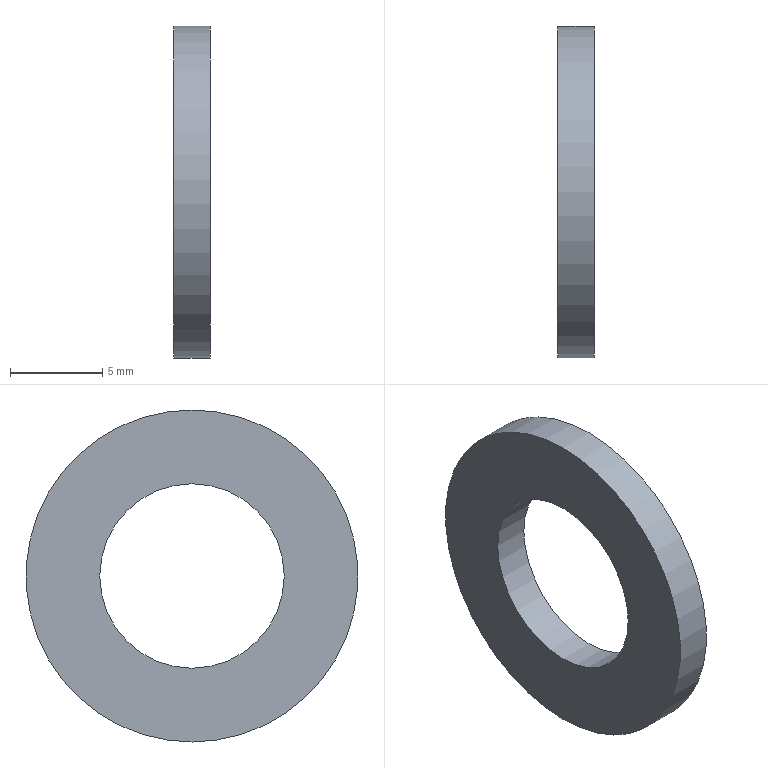Component | NX | CCJ-025 | 1 solid | 4 faces | box 2 x 18 x 18 mm | volume 352 mm3 | plane 2 | cylinder 2 | commonest cylinder face diameters 18 x1 10 x1
STEP:
#1=CARTESIAN_POINT('',(0.,0.,0.));
#2=DIRECTION('',(0.,0.,1.));
#3=DIRECTION('',(1.,0.,0.));
#4=AXIS2_PLACEMENT_3D('',#1,#2,#3);
#5=CARTESIAN_POINT('',(-40.,53.506,-47.227));
#6=VERTEX_POINT('',#5);
#7=CARTESIAN_POINT('',(-40.,53.506,-56.227));
#8=DIRECTION('',(-1.,0.,0.));
#9=DIRECTION('',(0.,0.,1.));
#10=AXIS2_PLACEMENT_3D('',#7,#8,#9);
#11=CIRCLE('',#10,9.);
#12=CARTESIAN_POINT('',(-40.,53.506,-56.227));
#13=DIRECTION('',(1.,0.,0.));
#14=DIRECTION('',(0.,0.,-1.));
#15=AXIS2_PLACEMENT_3D('',#12,#13,#14);
#16=PLANE('',#15);
#17=CARTESIAN_POINT('',(-9.,0.));
#18=CARTESIAN_POINT('',(-9.,15.588));
#19=CARTESIAN_POINT('',(4.5,7.794));
#20=CARTESIAN_POINT('',(18.,0.));
#21=CARTESIAN_POINT('',(4.5,-7.794));
#22=CARTESIAN_POINT('',(-9.,-15.588));
#23=CARTESIAN_POINT('',(-9.,0.));
#24=(BOUNDED_CURVE()B_SPLINE_CURVE(2,(#17,#18,#19,#20,#21,#22,#23),.UNSPECIFIED.,.T.,.F.)B_SPLINE_CURVE_WITH_KNOTS((1,2,2,2,2,1),(-2.094,0.,2.094,4.189,6.283,8.378),.UNSPECIFIED.)CURVE()GEOMETRIC_REPRESENTATION_ITEM()RATIONAL_B_SPLINE_CURVE((1.,0.5,1.,0.5,1.,0.5,1.))REPRESENTATION_ITEM(''));
#25=(GEOMETRIC_REPRESENTATION_CONTEXT(2)PARAMETRIC_REPRESENTATION_CONTEXT()REPRESENTATION_CONTEXT('',''));
#26=DEFINITIONAL_REPRESENTATION('',(#24),#25);
#27=PCURVE('',#16,#26);
#28=CARTESIAN_POINT('',(-40.,53.506,-56.227));
#29=DIRECTION('',(-1.,0.,0.));
#30=DIRECTION('',(0.,0.,1.));
#31=AXIS2_PLACEMENT_3D('',#28,#29,#30);
#32=CYLINDRICAL_SURFACE('',#31,9.);
#33=CARTESIAN_POINT('',(0.,0.));
#34=DIRECTION('',(1.,0.));
#35=VECTOR('',#34,1.);
#36=LINE('',#33,#35);
#37=(GEOMETRIC_REPRESENTATION_CONTEXT(2)PARAMETRIC_REPRESENTATION_CONTEXT()REPRESENTATION_CONTEXT('',''));
#38=DEFINITIONAL_REPRESENTATION('',(#36),#37);
#39=PCURVE('',#32,#38);
#40=SURFACE_CURVE('',#11,(#27,#39),.PCURVE_S1.);
#41=EDGE_CURVE('',#6,#6,#40,.T.);
#42=ORIENTED_EDGE('',*,*,#41,.F.);
#43=EDGE_LOOP('',(#42));
#44=FACE_BOUND('',#43,.T.);
#45=CARTESIAN_POINT('',(-40.,53.506,-51.227));
#46=VERTEX_POINT('',#45);
#47=CARTESIAN_POINT('',(-40.,53.506,-56.227));
#48=DIRECTION('',(-1.,0.,0.));
#49=DIRECTION('',(0.,0.,1.));
#50=AXIS2_PLACEMENT_3D('',#47,#48,#49);
#51=CIRCLE('',#50,5.);
#52=CARTESIAN_POINT('',(-5.,0.));
#53=CARTESIAN_POINT('',(-5.,8.66));
#54=CARTESIAN_POINT('',(2.5,4.33));
#55=CARTESIAN_POINT('',(10.,0.));
#56=CARTESIAN_POINT('',(2.5,-4.33));
#57=CARTESIAN_POINT('',(-5.,-8.66));
#58=CARTESIAN_POINT('',(-5.,0.));
#59=(BOUNDED_CURVE()B_SPLINE_CURVE(2,(#52,#53,#54,#55,#56,#57,#58),.UNSPECIFIED.,.T.,.F.)B_SPLINE_CURVE_WITH_KNOTS((1,2,2,2,2,1),(-2.094,0.,2.094,4.189,6.283,8.378),.UNSPECIFIED.)CURVE()GEOMETRIC_REPRESENTATION_ITEM()RATIONAL_B_SPLINE_CURVE((1.,0.5,1.,0.5,1.,0.5,1.))REPRESENTATION_ITEM(''));
#60=(GEOMETRIC_REPRESENTATION_CONTEXT(2)PARAMETRIC_REPRESENTATION_CONTEXT()REPRESENTATION_CONTEXT('',''));
#61=DEFINITIONAL_REPRESENTATION('',(#59),#60);
#62=PCURVE('',#16,#61);
#63=CARTESIAN_POINT('',(-40.,53.506,-56.227));
#64=DIRECTION('',(-1.,0.,0.));
#65=DIRECTION('',(0.,0.,1.));
#66=AXIS2_PLACEMENT_3D('',#63,#64,#65);
#67=CYLINDRICAL_SURFACE('',#66,5.);
#68=CARTESIAN_POINT('',(0.,0.));
#69=DIRECTION('',(1.,0.));
#70=VECTOR('',#69,1.);
#71=LINE('',#68,#70);
#72=(GEOMETRIC_REPRESENTATION_CONTEXT(2)PARAMETRIC_REPRESENTATION_CONTEXT()REPRESENTATION_CONTEXT('',''));
#73=DEFINITIONAL_REPRESENTATION('',(#71),#72);
#74=PCURVE('',#67,#73);
#75=SURFACE_CURVE('',#51,(#62,#74),.PCURVE_S1.);
#76=EDGE_CURVE('',#46,#46,#75,.T.);
#77=ORIENTED_EDGE('',*,*,#76,.T.);
#78=EDGE_LOOP('',(#77));
#79=FACE_BOUND('',#78,.T.);
#80=ADVANCED_FACE('',(#44,#79),#16,.T.);
#81=CARTESIAN_POINT('',(-42.,53.506,-47.227));
#82=VERTEX_POINT('',#81);
#83=CARTESIAN_POINT('',(-42.,53.506,-56.227));
#84=DIRECTION('',(-1.,0.,0.));
#85=DIRECTION('',(0.,0.,1.));
#86=AXIS2_PLACEMENT_3D('',#83,#84,#85);
#87=CIRCLE('',#86,9.);
#88=CARTESIAN_POINT('',(-42.,53.506,-56.227));
#89=DIRECTION('',(1.,0.,0.));
#90=DIRECTION('',(0.,0.,-1.));
#91=AXIS2_PLACEMENT_3D('',#88,#89,#90);
#92=PLANE('',#91);
#93=CARTESIAN_POINT('',(-9.,0.));
#94=CARTESIAN_POINT('',(-9.,15.588));
#95=CARTESIAN_POINT('',(4.5,7.794));
#96=CARTESIAN_POINT('',(18.,0.));
#97=CARTESIAN_POINT('',(4.5,-7.794));
#98=CARTESIAN_POINT('',(-9.,-15.588));
#99=CARTESIAN_POINT('',(-9.,0.));
#100=(BOUNDED_CURVE()B_SPLINE_CURVE(2,(#93,#94,#95,#96,#97,#98,#99),.UNSPECIFIED.,.T.,.F.)B_SPLINE_CURVE_WITH_KNOTS((1,2,2,2,2,1),(-2.094,0.,2.094,4.189,6.283,8.378),.UNSPECIFIED.)CURVE()GEOMETRIC_REPRESENTATION_ITEM()RATIONAL_B_SPLINE_CURVE((1.,0.5,1.,0.5,1.,0.5,1.))REPRESENTATION_ITEM(''));
#101=(GEOMETRIC_REPRESENTATION_CONTEXT(2)PARAMETRIC_REPRESENTATION_CONTEXT()REPRESENTATION_CONTEXT('',''));
#102=DEFINITIONAL_REPRESENTATION('',(#100),#101);
#103=PCURVE('',#92,#102);
#104=CARTESIAN_POINT('',(0.,2.));
#105=DIRECTION('',(1.,0.));
#106=VECTOR('',#105,1.);
#107=LINE('',#104,#106);
#108=(GEOMETRIC_REPRESENTATION_CONTEXT(2)PARAMETRIC_REPRESENTATION_CONTEXT()REPRESENTATION_CONTEXT('',''));
#109=DEFINITIONAL_REPRESENTATION('',(#107),#108);
#110=PCURVE('',#32,#109);
#111=SURFACE_CURVE('',#87,(#103,#110),.PCURVE_S1.);
#112=EDGE_CURVE('',#82,#82,#111,.T.);
#113=ORIENTED_EDGE('',*,*,#112,.T.);
#114=EDGE_LOOP('',(#113));
#115=FACE_BOUND('',#114,.T.);
#116=CARTESIAN_POINT('',(-42.,53.506,-51.227));
#117=VERTEX_POINT('',#116);
#118=CARTESIAN_POINT('',(-42.,53.506,-56.227));
#119=DIRECTION('',(-1.,0.,0.));
#120=DIRECTION('',(0.,0.,1.));
#121=AXIS2_PLACEMENT_3D('',#118,#119,#120);
#122=CIRCLE('',#121,5.);
#123=CARTESIAN_POINT('',(-5.,0.));
#124=CARTESIAN_POINT('',(-5.,8.66));
#125=CARTESIAN_POINT('',(2.5,4.33));
#126=CARTESIAN_POINT('',(10.,0.));
#127=CARTESIAN_POINT('',(2.5,-4.33));
#128=CARTESIAN_POINT('',(-5.,-8.66));
#129=CARTESIAN_POINT('',(-5.,0.));
#130=(BOUNDED_CURVE()B_SPLINE_CURVE(2,(#123,#124,#125,#126,#127,#128,#129),.UNSPECIFIED.,.T.,.F.)B_SPLINE_CURVE_WITH_KNOTS((1,2,2,2,2,1),(-2.094,0.,2.094,4.189,6.283,8.378),.UNSPECIFIED.)CURVE()GEOMETRIC_REPRESENTATION_ITEM()RATIONAL_B_SPLINE_CURVE((1.,0.5,1.,0.5,1.,0.5,1.))REPRESENTATION_ITEM(''));
#131=(GEOMETRIC_REPRESENTATION_CONTEXT(2)PARAMETRIC_REPRESENTATION_CONTEXT()REPRESENTATION_CONTEXT('',''));
#132=DEFINITIONAL_REPRESENTATION('',(#130),#131);
#133=PCURVE('',#92,#132);
#134=CARTESIAN_POINT('',(0.,2.));
#135=DIRECTION('',(1.,0.));
#136=VECTOR('',#135,1.);
#137=LINE('',#134,#136);
#138=(GEOMETRIC_REPRESENTATION_CONTEXT(2)PARAMETRIC_REPRESENTATION_CONTEXT()REPRESENTATION_CONTEXT('',''));
#139=DEFINITIONAL_REPRESENTATION('',(#137),#138);
#140=PCURVE('',#67,#139);
#141=SURFACE_CURVE('',#122,(#133,#140),.PCURVE_S1.);
#142=EDGE_CURVE('',#117,#117,#141,.T.);
#143=ORIENTED_EDGE('',*,*,#142,.F.);
#144=EDGE_LOOP('',(#143));
#145=FACE_BOUND('',#144,.T.);
#146=ADVANCED_FACE('',(#115,#145),#92,.F.);
#147=ORIENTED_EDGE('',*,*,#41,.T.);
#148=CARTESIAN_POINT('',(-40.,53.506,-47.227));
#149=CARTESIAN_POINT('',(-42.,53.506,-47.227));
#150=B_SPLINE_CURVE_WITH_KNOTS('',1,(#148,#149),.UNSPECIFIED.,.F.,.F.,(2,2),(0.,2.),.PIECEWISE_BEZIER_KNOTS.);
#151=CARTESIAN_POINT('',(6.283,0.));
#152=DIRECTION('',(0.,1.));
#153=VECTOR('',#152,1.);
#154=LINE('',#151,#153);
#155=(GEOMETRIC_REPRESENTATION_CONTEXT(2)PARAMETRIC_REPRESENTATION_CONTEXT()REPRESENTATION_CONTEXT('',''));
#156=DEFINITIONAL_REPRESENTATION('',(#154),#155);
#157=PCURVE('',#32,#156);
#158=CARTESIAN_POINT('',(0.,0.));
#159=DIRECTION('',(0.,1.));
#160=VECTOR('',#159,1.);
#161=LINE('',#158,#160);
#162=(GEOMETRIC_REPRESENTATION_CONTEXT(2)PARAMETRIC_REPRESENTATION_CONTEXT()REPRESENTATION_CONTEXT('',''));
#163=DEFINITIONAL_REPRESENTATION('',(#161),#162);
#164=PCURVE('',#32,#163);
#165=SEAM_CURVE('',#150,(#157,#164),.PCURVE_S1.);
#166=EDGE_CURVE('',#6,#82,#165,.T.);
#167=ORIENTED_EDGE('',*,*,#166,.T.);
#168=ORIENTED_EDGE('',*,*,#112,.F.);
#169=ORIENTED_EDGE('',*,*,#166,.F.);
#170=EDGE_LOOP('',(#147,#167,#168,#169));
#171=FACE_BOUND('',#170,.T.);
#172=ADVANCED_FACE('',(#171),#32,.T.);
#173=ORIENTED_EDGE('',*,*,#76,.T.);
#174=CARTESIAN_POINT('',(-40.,53.506,-51.227));
#175=CARTESIAN_POINT('',(-42.,53.506,-51.227));
#176=B_SPLINE_CURVE_WITH_KNOTS('',1,(#174,#175),.UNSPECIFIED.,.F.,.F.,(2,2),(0.,2.),.PIECEWISE_BEZIER_KNOTS.);
#177=CARTESIAN_POINT('',(6.283,0.));
#178=DIRECTION('',(0.,1.));
#179=VECTOR('',#178,1.);
#180=LINE('',#177,#179);
#181=(GEOMETRIC_REPRESENTATION_CONTEXT(2)PARAMETRIC_REPRESENTATION_CONTEXT()REPRESENTATION_CONTEXT('',''));
#182=DEFINITIONAL_REPRESENTATION('',(#180),#181);
#183=PCURVE('',#67,#182);
#184=CARTESIAN_POINT('',(0.,0.));
#185=DIRECTION('',(0.,1.));
#186=VECTOR('',#185,1.);
#187=LINE('',#184,#186);
#188=(GEOMETRIC_REPRESENTATION_CONTEXT(2)PARAMETRIC_REPRESENTATION_CONTEXT()REPRESENTATION_CONTEXT('',''));
#189=DEFINITIONAL_REPRESENTATION('',(#187),#188);
#190=PCURVE('',#67,#189);
#191=SEAM_CURVE('',#176,(#183,#190),.PCURVE_S1.);
#192=EDGE_CURVE('',#46,#117,#191,.T.);
#193=ORIENTED_EDGE('',*,*,#192,.T.);
#194=ORIENTED_EDGE('',*,*,#142,.F.);
#195=ORIENTED_EDGE('',*,*,#192,.F.);
#196=EDGE_LOOP('',(#173,#193,#194,#195));
#197=FACE_BOUND('',#196,.F.);
#198=ADVANCED_FACE('',(#197),#67,.F.);
#199=CLOSED_SHELL('',(#80,#146,#172,#198));
#200=MANIFOLD_SOLID_BREP('',#199);
#201=(LENGTH_UNIT()NAMED_UNIT(*)SI_UNIT(.MILLI.,.METRE.));
#202=UNCERTAINTY_MEASURE_WITH_UNIT(LENGTH_MEASURE(0.00001),#201,'','');
#203=(NAMED_UNIT(*)PLANE_ANGLE_UNIT()SI_UNIT($,.RADIAN.));
#204=(NAMED_UNIT(*)SI_UNIT($,.STERADIAN.)SOLID_ANGLE_UNIT());
#205=(GEOMETRIC_REPRESENTATION_CONTEXT(3)GLOBAL_UNCERTAINTY_ASSIGNED_CONTEXT((#202))GLOBAL_UNIT_ASSIGNED_CONTEXT((#201,#203,#204))REPRESENTATION_CONTEXT('',''));
#206=ADVANCED_BREP_SHAPE_REPRESENTATION('',(#4,#200),#205);